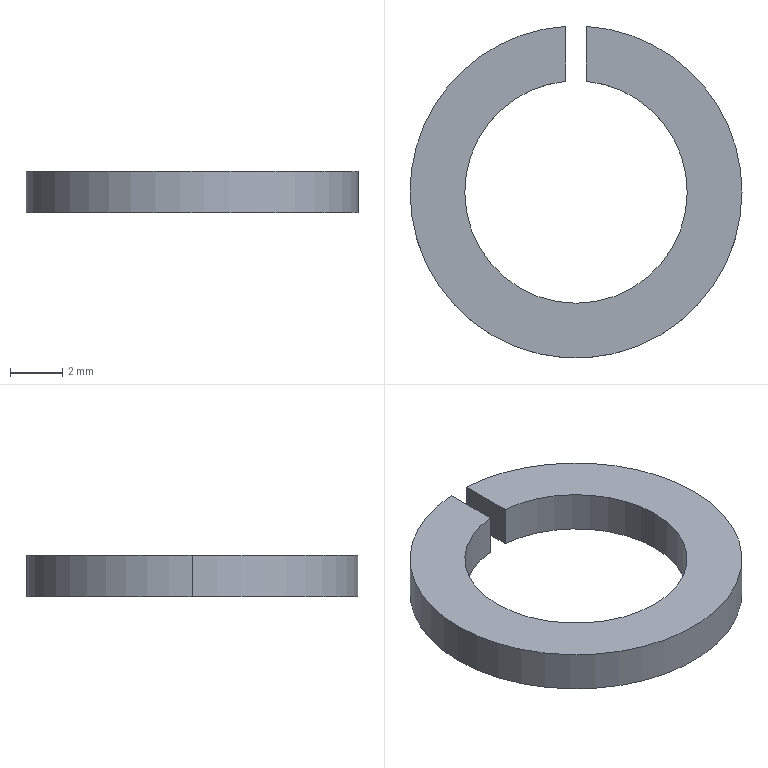Component | SolidWorks | GB_T93-1987StandardTypeSpringWasher(Assembly)8x2.1-5 | 1 solid | 10 faces | box 12.69 x 12.67 x 1.6 mm | volume 109 mm3 | cylinder 6 | plane 4 | commonest cylinder face diameters 8.5 x3 12.688 x3
build123d program:
from build123d import *

# Parameters (mm, degrees)
EXTRUDE1_DEPTH = 1.6


with BuildPart() as part:
    # Sketch1 → Extrude1 (new body)
    with BuildSketch(Plane.XY):
        with BuildLine():
            Line((-0.4, 6.331), (-0.4, 4.231))
            ThreePointArc((-0.4, 4.231), (0, -4.25), (0.4, 4.231))
            Line((0.4, 4.231), (0.4, 6.331))
            ThreePointArc((0.4, 6.331), (0, -6.344), (-0.4, 6.331))
        make_face()
    extrude(amount=EXTRUDE1_DEPTH)


solid = part.part

# Placed as in the assembly
solid = solid.moved(Location((280, -19, -38.2), (0, 0, 0)))
STEP:
#1=COLOUR_RGB('',0.7922,0.8196,0.9333);
#2=FILL_AREA_STYLE_COLOUR('',#1);
#3=FILL_AREA_STYLE('',(#2));
#4=SURFACE_STYLE_FILL_AREA(#3);
#5=SURFACE_SIDE_STYLE('',(#4));
#6=SURFACE_STYLE_USAGE(.BOTH.,#5);
#7=PRESENTATION_STYLE_ASSIGNMENT((#6));
#8=CARTESIAN_POINT('',(11.191,-0.748,-1.441));
#9=VERTEX_POINT('',#8);
#10=CARTESIAN_POINT('',(10.856,-0.748,-1.441));
#11=VERTEX_POINT('',#10);
#12=CARTESIAN_POINT('',(11.024,-0.748,-1.441));
#13=DIRECTION('',(0.,0.,-1.));
#14=DIRECTION('',(1.,0.,0.));
#15=AXIS2_PLACEMENT_3D('',#12,#13,#14);
#16=CIRCLE('',#15,0.1673);
#17=EDGE_CURVE('',#9,#11,#16,.T.);
#18=ORIENTED_EDGE('',*,*,#17,.F.);
#19=CARTESIAN_POINT('',(11.191,-0.748,-1.504));
#20=VERTEX_POINT('',#19);
#21=CARTESIAN_POINT('',(11.191,-0.748,-1.441));
#22=DIRECTION('',(0.,0.,-1.));
#23=VECTOR('',#22,39.37);
#24=LINE('',#21,#23);
#25=EDGE_CURVE('',#9,#20,#24,.T.);
#26=ORIENTED_EDGE('',*,*,#25,.T.);
#27=CARTESIAN_POINT('',(10.856,-0.748,-1.504));
#28=VERTEX_POINT('',#27);
#29=CARTESIAN_POINT('',(11.024,-0.748,-1.504));
#30=DIRECTION('',(0.,0.,-1.));
#31=DIRECTION('',(1.,0.,0.));
#32=AXIS2_PLACEMENT_3D('',#29,#30,#31);
#33=CIRCLE('',#32,0.1673);
#34=EDGE_CURVE('',#20,#28,#33,.T.);
#35=ORIENTED_EDGE('',*,*,#34,.T.);
#36=CARTESIAN_POINT('',(10.856,-0.748,-1.441));
#37=DIRECTION('',(0.,0.,-1.));
#38=VECTOR('',#37,39.37);
#39=LINE('',#36,#38);
#40=EDGE_CURVE('',#11,#28,#39,.T.);
#41=ORIENTED_EDGE('',*,*,#40,.F.);
#42=EDGE_LOOP('',(#18,#26,#35,#41));
#43=FACE_OUTER_BOUND('',#42,.T.);
#44=CARTESIAN_POINT('',(11.024,-0.748,-1.441));
#45=DIRECTION('',(0.,0.,-1.));
#46=DIRECTION('',(-1.,0.,0.));
#47=AXIS2_PLACEMENT_3D('',#44,#45,#46);
#48=CYLINDRICAL_SURFACE('',#47,0.1673);
#49=ADVANCED_FACE('',(#43),#48,.F.);
#50=CARTESIAN_POINT('',(11.008,-0.5815,-1.441));
#51=VERTEX_POINT('',#50);
#52=CARTESIAN_POINT('',(11.024,-0.748,-1.441));
#53=DIRECTION('',(0.,0.,-1.));
#54=DIRECTION('',(1.,0.,0.));
#55=AXIS2_PLACEMENT_3D('',#52,#53,#54);
#56=CIRCLE('',#55,0.1673);
#57=EDGE_CURVE('',#11,#51,#56,.T.);
#58=ORIENTED_EDGE('',*,*,#57,.F.);
#59=ORIENTED_EDGE('',*,*,#40,.T.);
#60=CARTESIAN_POINT('',(11.008,-0.5815,-1.504));
#61=VERTEX_POINT('',#60);
#62=CARTESIAN_POINT('',(11.024,-0.748,-1.504));
#63=DIRECTION('',(0.,0.,-1.));
#64=DIRECTION('',(1.,0.,0.));
#65=AXIS2_PLACEMENT_3D('',#62,#63,#64);
#66=CIRCLE('',#65,0.1673);
#67=EDGE_CURVE('',#28,#61,#66,.T.);
#68=ORIENTED_EDGE('',*,*,#67,.T.);
#69=CARTESIAN_POINT('',(11.008,-0.5815,-1.441));
#70=DIRECTION('',(0.,0.,-1.));
#71=VECTOR('',#70,39.37);
#72=LINE('',#69,#71);
#73=EDGE_CURVE('',#51,#61,#72,.T.);
#74=ORIENTED_EDGE('',*,*,#73,.F.);
#75=EDGE_LOOP('',(#58,#59,#68,#74));
#76=FACE_OUTER_BOUND('',#75,.T.);
#77=CARTESIAN_POINT('',(11.024,-0.748,-1.441));
#78=DIRECTION('',(0.,0.,-1.));
#79=DIRECTION('',(-1.,0.,0.));
#80=AXIS2_PLACEMENT_3D('',#77,#78,#79);
#81=CYLINDRICAL_SURFACE('',#80,0.1673);
#82=ADVANCED_FACE('',(#76),#81,.F.);
#83=CARTESIAN_POINT('',(11.273,-0.748,-1.441));
#84=VERTEX_POINT('',#83);
#85=CARTESIAN_POINT('',(11.039,-0.4988,-1.441));
#86=VERTEX_POINT('',#85);
#87=CARTESIAN_POINT('',(11.024,-0.748,-1.441));
#88=DIRECTION('',(0.,0.,1.));
#89=DIRECTION('',(1.,0.,0.));
#90=AXIS2_PLACEMENT_3D('',#87,#88,#89);
#91=CIRCLE('',#90,0.2498);
#92=EDGE_CURVE('',#84,#86,#91,.T.);
#93=ORIENTED_EDGE('',*,*,#92,.F.);
#94=CARTESIAN_POINT('',(11.273,-0.748,-1.504));
#95=VERTEX_POINT('',#94);
#96=CARTESIAN_POINT('',(11.273,-0.748,-1.441));
#97=DIRECTION('',(0.,0.,-1.));
#98=VECTOR('',#97,39.37);
#99=LINE('',#96,#98);
#100=EDGE_CURVE('',#84,#95,#99,.T.);
#101=ORIENTED_EDGE('',*,*,#100,.T.);
#102=CARTESIAN_POINT('',(11.039,-0.4988,-1.504));
#103=VERTEX_POINT('',#102);
#104=CARTESIAN_POINT('',(11.024,-0.748,-1.504));
#105=DIRECTION('',(0.,0.,1.));
#106=DIRECTION('',(1.,0.,0.));
#107=AXIS2_PLACEMENT_3D('',#104,#105,#106);
#108=CIRCLE('',#107,0.2498);
#109=EDGE_CURVE('',#95,#103,#108,.T.);
#110=ORIENTED_EDGE('',*,*,#109,.T.);
#111=CARTESIAN_POINT('',(11.039,-0.4988,-1.441));
#112=DIRECTION('',(0.,0.,-1.));
#113=VECTOR('',#112,39.37);
#114=LINE('',#111,#113);
#115=EDGE_CURVE('',#86,#103,#114,.T.);
#116=ORIENTED_EDGE('',*,*,#115,.F.);
#117=EDGE_LOOP('',(#93,#101,#110,#116));
#118=FACE_OUTER_BOUND('',#117,.T.);
#119=CARTESIAN_POINT('',(11.024,-0.748,-1.441));
#120=DIRECTION('',(0.,0.,-1.));
#121=DIRECTION('',(-1.,0.,0.));
#122=AXIS2_PLACEMENT_3D('',#119,#120,#121);
#123=CYLINDRICAL_SURFACE('',#122,0.2498);
#124=ADVANCED_FACE('',(#118),#123,.T.);
#125=ORIENTED_EDGE('',*,*,#100,.F.);
#126=CARTESIAN_POINT('',(10.774,-0.748,-1.441));
#127=VERTEX_POINT('',#126);
#128=CARTESIAN_POINT('',(11.024,-0.748,-1.441));
#129=DIRECTION('',(0.,0.,1.));
#130=DIRECTION('',(1.,0.,0.));
#131=AXIS2_PLACEMENT_3D('',#128,#129,#130);
#132=CIRCLE('',#131,0.2498);
#133=EDGE_CURVE('',#127,#84,#132,.T.);
#134=ORIENTED_EDGE('',*,*,#133,.F.);
#135=CARTESIAN_POINT('',(10.774,-0.748,-1.504));
#136=VERTEX_POINT('',#135);
#137=CARTESIAN_POINT('',(10.774,-0.748,-1.441));
#138=DIRECTION('',(0.,0.,-1.));
#139=VECTOR('',#138,39.37);
#140=LINE('',#137,#139);
#141=EDGE_CURVE('',#127,#136,#140,.T.);
#142=ORIENTED_EDGE('',*,*,#141,.T.);
#143=CARTESIAN_POINT('',(11.024,-0.748,-1.504));
#144=DIRECTION('',(0.,0.,1.));
#145=DIRECTION('',(1.,0.,0.));
#146=AXIS2_PLACEMENT_3D('',#143,#144,#145);
#147=CIRCLE('',#146,0.2498);
#148=EDGE_CURVE('',#136,#95,#147,.T.);
#149=ORIENTED_EDGE('',*,*,#148,.T.);
#150=EDGE_LOOP('',(#125,#134,#142,#149));
#151=FACE_OUTER_BOUND('',#150,.T.);
#152=CARTESIAN_POINT('',(11.024,-0.748,-1.441));
#153=DIRECTION('',(0.,0.,-1.));
#154=DIRECTION('',(-1.,0.,0.));
#155=AXIS2_PLACEMENT_3D('',#152,#153,#154);
#156=CYLINDRICAL_SURFACE('',#155,0.2498);
#157=ADVANCED_FACE('',(#151),#156,.T.);
#158=ORIENTED_EDGE('',*,*,#141,.F.);
#159=CARTESIAN_POINT('',(11.008,-0.4988,-1.441));
#160=VERTEX_POINT('',#159);
#161=CARTESIAN_POINT('',(11.024,-0.748,-1.441));
#162=DIRECTION('',(0.,0.,1.));
#163=DIRECTION('',(1.,0.,0.));
#164=AXIS2_PLACEMENT_3D('',#161,#162,#163);
#165=CIRCLE('',#164,0.2498);
#166=EDGE_CURVE('',#160,#127,#165,.T.);
#167=ORIENTED_EDGE('',*,*,#166,.F.);
#168=CARTESIAN_POINT('',(11.008,-0.4988,-1.504));
#169=VERTEX_POINT('',#168);
#170=CARTESIAN_POINT('',(11.008,-0.4988,-1.441));
#171=DIRECTION('',(0.,0.,-1.));
#172=VECTOR('',#171,39.37);
#173=LINE('',#170,#172);
#174=EDGE_CURVE('',#160,#169,#173,.T.);
#175=ORIENTED_EDGE('',*,*,#174,.T.);
#176=CARTESIAN_POINT('',(11.024,-0.748,-1.504));
#177=DIRECTION('',(0.,0.,1.));
#178=DIRECTION('',(1.,0.,0.));
#179=AXIS2_PLACEMENT_3D('',#176,#177,#178);
#180=CIRCLE('',#179,0.2498);
#181=EDGE_CURVE('',#169,#136,#180,.T.);
#182=ORIENTED_EDGE('',*,*,#181,.T.);
#183=EDGE_LOOP('',(#158,#167,#175,#182));
#184=FACE_OUTER_BOUND('',#183,.T.);
#185=CARTESIAN_POINT('',(11.024,-0.748,-1.441));
#186=DIRECTION('',(0.,0.,-1.));
#187=DIRECTION('',(-1.,0.,0.));
#188=AXIS2_PLACEMENT_3D('',#185,#186,#187);
#189=CYLINDRICAL_SURFACE('',#188,0.2498);
#190=ADVANCED_FACE('',(#184),#189,.T.);
#191=CARTESIAN_POINT('',(11.039,-0.5815,-1.504));
#192=VERTEX_POINT('',#191);
#193=CARTESIAN_POINT('',(11.039,-0.4988,-1.504));
#194=DIRECTION('',(0.,-1.,0.));
#195=VECTOR('',#194,39.37);
#196=LINE('',#193,#195);
#197=EDGE_CURVE('',#103,#192,#196,.T.);
#198=ORIENTED_EDGE('',*,*,#197,.T.);
#199=CARTESIAN_POINT('',(11.039,-0.5815,-1.441));
#200=VERTEX_POINT('',#199);
#201=CARTESIAN_POINT('',(11.039,-0.5815,-1.441));
#202=DIRECTION('',(0.,0.,-1.));
#203=VECTOR('',#202,39.37);
#204=LINE('',#201,#203);
#205=EDGE_CURVE('',#200,#192,#204,.T.);
#206=ORIENTED_EDGE('',*,*,#205,.F.);
#207=CARTESIAN_POINT('',(11.039,-0.4988,-1.441));
#208=DIRECTION('',(0.,-1.,0.));
#209=VECTOR('',#208,39.37);
#210=LINE('',#207,#209);
#211=EDGE_CURVE('',#86,#200,#210,.T.);
#212=ORIENTED_EDGE('',*,*,#211,.F.);
#213=ORIENTED_EDGE('',*,*,#115,.T.);
#214=EDGE_LOOP('',(#198,#206,#212,#213));
#215=FACE_OUTER_BOUND('',#214,.T.);
#216=CARTESIAN_POINT('',(11.039,-0.4988,-1.441));
#217=DIRECTION('',(1.,0.,0.));
#218=DIRECTION('',(-0.,1.,0.));
#219=AXIS2_PLACEMENT_3D('',#216,#217,#218);
#220=PLANE('',#219);
#221=ADVANCED_FACE('',(#215),#220,.F.);
#222=ORIENTED_EDGE('',*,*,#25,.F.);
#223=CARTESIAN_POINT('',(11.024,-0.748,-1.441));
#224=DIRECTION('',(0.,0.,-1.));
#225=DIRECTION('',(1.,0.,0.));
#226=AXIS2_PLACEMENT_3D('',#223,#224,#225);
#227=CIRCLE('',#226,0.1673);
#228=EDGE_CURVE('',#200,#9,#227,.T.);
#229=ORIENTED_EDGE('',*,*,#228,.F.);
#230=ORIENTED_EDGE('',*,*,#205,.T.);
#231=CARTESIAN_POINT('',(11.024,-0.748,-1.504));
#232=DIRECTION('',(0.,0.,-1.));
#233=DIRECTION('',(1.,0.,0.));
#234=AXIS2_PLACEMENT_3D('',#231,#232,#233);
#235=CIRCLE('',#234,0.1673);
#236=EDGE_CURVE('',#192,#20,#235,.T.);
#237=ORIENTED_EDGE('',*,*,#236,.T.);
#238=EDGE_LOOP('',(#222,#229,#230,#237));
#239=FACE_OUTER_BOUND('',#238,.T.);
#240=CARTESIAN_POINT('',(11.024,-0.748,-1.441));
#241=DIRECTION('',(0.,0.,-1.));
#242=DIRECTION('',(-1.,0.,0.));
#243=AXIS2_PLACEMENT_3D('',#240,#241,#242);
#244=CYLINDRICAL_SURFACE('',#243,0.1673);
#245=ADVANCED_FACE('',(#239),#244,.F.);
#246=CARTESIAN_POINT('',(11.008,-0.4988,-1.504));
#247=DIRECTION('',(-0.,1.,0.));
#248=VECTOR('',#247,39.37);
#249=LINE('',#246,#248);
#250=EDGE_CURVE('',#61,#169,#249,.T.);
#251=ORIENTED_EDGE('',*,*,#250,.T.);
#252=ORIENTED_EDGE('',*,*,#174,.F.);
#253=CARTESIAN_POINT('',(11.008,-0.4988,-1.441));
#254=DIRECTION('',(-0.,1.,0.));
#255=VECTOR('',#254,39.37);
#256=LINE('',#253,#255);
#257=EDGE_CURVE('',#51,#160,#256,.T.);
#258=ORIENTED_EDGE('',*,*,#257,.F.);
#259=ORIENTED_EDGE('',*,*,#73,.T.);
#260=EDGE_LOOP('',(#251,#252,#258,#259));
#261=FACE_OUTER_BOUND('',#260,.T.);
#262=CARTESIAN_POINT('',(11.008,-0.4988,-1.441));
#263=DIRECTION('',(-1.,-0.,0.));
#264=DIRECTION('',(0.,-1.,0.));
#265=AXIS2_PLACEMENT_3D('',#262,#263,#264);
#266=PLANE('',#265);
#267=ADVANCED_FACE('',(#261),#266,.F.);
#268=ORIENTED_EDGE('',*,*,#166,.T.);
#269=ORIENTED_EDGE('',*,*,#133,.T.);
#270=ORIENTED_EDGE('',*,*,#92,.T.);
#271=ORIENTED_EDGE('',*,*,#211,.T.);
#272=ORIENTED_EDGE('',*,*,#228,.T.);
#273=ORIENTED_EDGE('',*,*,#17,.T.);
#274=ORIENTED_EDGE('',*,*,#57,.T.);
#275=ORIENTED_EDGE('',*,*,#257,.T.);
#276=EDGE_LOOP('',(#268,#269,#270,#271,#272,#273,#274,#275));
#277=FACE_OUTER_BOUND('',#276,.T.);
#278=CARTESIAN_POINT('',(11.024,-0.748,-1.441));
#279=DIRECTION('',(0.,0.,1.));
#280=DIRECTION('',(1.,0.,0.));
#281=AXIS2_PLACEMENT_3D('',#278,#279,#280);
#282=PLANE('',#281);
#283=ADVANCED_FACE('',(#277),#282,.T.);
#284=ORIENTED_EDGE('',*,*,#181,.F.);
#285=ORIENTED_EDGE('',*,*,#250,.F.);
#286=ORIENTED_EDGE('',*,*,#67,.F.);
#287=ORIENTED_EDGE('',*,*,#34,.F.);
#288=ORIENTED_EDGE('',*,*,#236,.F.);
#289=ORIENTED_EDGE('',*,*,#197,.F.);
#290=ORIENTED_EDGE('',*,*,#109,.F.);
#291=ORIENTED_EDGE('',*,*,#148,.F.);
#292=EDGE_LOOP('',(#284,#285,#286,#287,#288,#289,#290,#291));
#293=FACE_OUTER_BOUND('',#292,.T.);
#294=CARTESIAN_POINT('',(11.024,-0.748,-1.504));
#295=DIRECTION('',(0.,0.,1.));
#296=DIRECTION('',(1.,0.,0.));
#297=AXIS2_PLACEMENT_3D('',#294,#295,#296);
#298=PLANE('',#297);
#299=ADVANCED_FACE('',(#293),#298,.F.);
#300=CLOSED_SHELL('',(#49,#82,#124,#157,#190,#221,#245,#267,#283,#299));
#301=MANIFOLD_SOLID_BREP('',#300);
#302=STYLED_ITEM('',(#7),#301);
#303=(LENGTH_UNIT()NAMED_UNIT(*)SI_UNIT($,.METRE.));
#304=LENGTH_MEASURE_WITH_UNIT(LENGTH_MEASURE(0.0254),#303);
#305=DIMENSIONAL_EXPONENTS(1.,0.,0.,0.,0.,0.,0.);
#306=(CONVERSION_BASED_UNIT('',#304)LENGTH_UNIT()NAMED_UNIT(#305));
#307=UNCERTAINTY_MEASURE_WITH_UNIT(LENGTH_MEASURE(0.00001),#306,'','');
#308=(NAMED_UNIT(*)PLANE_ANGLE_UNIT()SI_UNIT($,.RADIAN.));
#309=(NAMED_UNIT(*)SI_UNIT($,.STERADIAN.)SOLID_ANGLE_UNIT());
#310=(GEOMETRIC_REPRESENTATION_CONTEXT(3)GLOBAL_UNCERTAINTY_ASSIGNED_CONTEXT((#307))GLOBAL_UNIT_ASSIGNED_CONTEXT((#306,#308,#309))REPRESENTATION_CONTEXT('',''));
#311=MECHANICAL_DESIGN_GEOMETRIC_PRESENTATION_REPRESENTATION('',(#302),#310);
#312=PRESENTATION_LAYER_ASSIGNMENT('','',(#302));
#313=CARTESIAN_POINT('',(0.,0.,0.));
#314=DIRECTION('',(0.,0.,1.));
#315=DIRECTION('',(1.,0.,0.));
#316=AXIS2_PLACEMENT_3D('',#313,#314,#315);
#317=(LENGTH_UNIT()NAMED_UNIT(*)SI_UNIT($,.METRE.));
#318=LENGTH_MEASURE_WITH_UNIT(LENGTH_MEASURE(0.0254),#317);
#319=DIMENSIONAL_EXPONENTS(1.,0.,0.,0.,0.,0.,0.);
#320=(CONVERSION_BASED_UNIT('',#318)LENGTH_UNIT()NAMED_UNIT(#319));
#321=UNCERTAINTY_MEASURE_WITH_UNIT(LENGTH_MEASURE(0.00001),#320,'','');
#322=(NAMED_UNIT(*)PLANE_ANGLE_UNIT()SI_UNIT($,.RADIAN.));
#323=(NAMED_UNIT(*)SI_UNIT($,.STERADIAN.)SOLID_ANGLE_UNIT());
#324=(GEOMETRIC_REPRESENTATION_CONTEXT(3)GLOBAL_UNCERTAINTY_ASSIGNED_CONTEXT((#321))GLOBAL_UNIT_ASSIGNED_CONTEXT((#320,#322,#323))REPRESENTATION_CONTEXT('',''));
#325=ADVANCED_BREP_SHAPE_REPRESENTATION('',(#301,#316),#324);